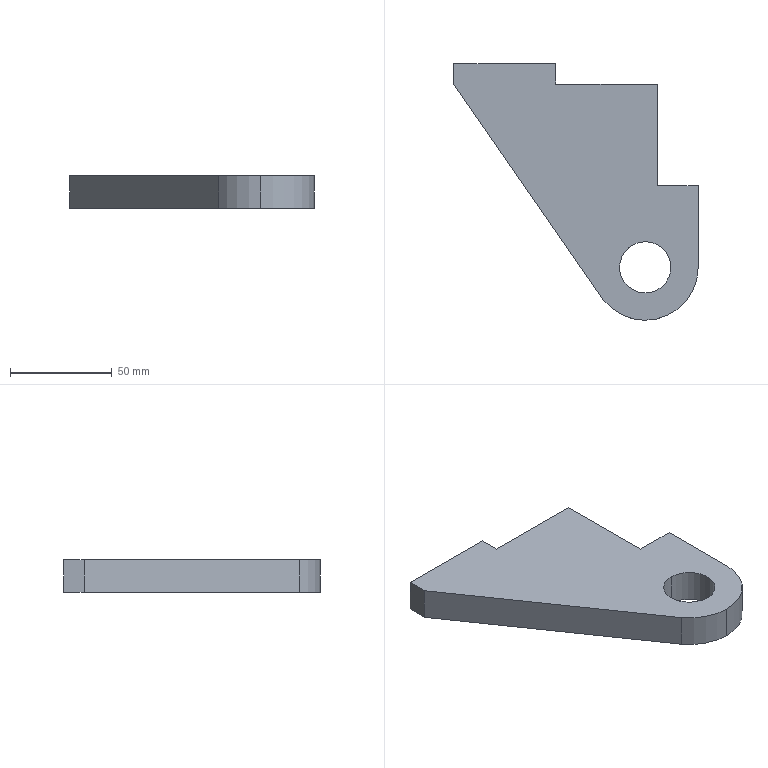Component | SolidWorks | VehicleBodyUpperLug-2 | 1 solid | 14 faces | box 120 x 126 x 16 mm | volume 129354 mm3 | plane 10 | cylinder 4 | commonest cylinder face diameters 25.2 x2 52 x2 | material Q235
build123d program:
from build123d import *

# Parameters (mm, degrees)
SKETCH1_R           = 12.6
BOSS_EXTRUDE1_DEPTH = 16


with BuildPart() as part:
    # Sketch1 → Boss-Extrude1 (new body)
    with BuildSketch(Plane.XY):
        with BuildLine():
            Line((96.756, 48.198), (133.752, 48.562))
            Line((133.752, 48.562), (133.556, 68.561))
            Line((133.556, 68.561), (183.553, 69.052))
            Line((183.553, 69.052), (183.259, 99.05))
            Line((183.259, 99.05), (183.062, 119.049))
            Line((183.062, 119.049), (193.062, 119.147))
            Line((193.062, 119.147), (192.571, 169.145))
            Line((192.571, 169.145), (182.571, 169.047))
            Line((182.571, 169.047), (77.704, 94.818))
            ThreePointArc((77.704, 94.818), (68.916, 65.708), (93.756, 48.169))
            Line((93.756, 48.169), (96.756, 48.198))
        make_face()
        with Locations((93.501, 74.168)):
            Circle(SKETCH1_R, mode=Mode.SUBTRACT)
    extrude(amount=BOSS_EXTRUDE1_DEPTH)


solid = part.part

# Placed as in the assembly
solid = solid.moved(Location((-209.351, 1092.251, 2619.537), (0, 0, 89.437)))
STEP:
#1=COLOUR_RGB('',0.7922,0.8196,0.9333);
#2=FILL_AREA_STYLE_COLOUR('',#1);
#3=FILL_AREA_STYLE('',(#2));
#4=SURFACE_STYLE_FILL_AREA(#3);
#5=SURFACE_SIDE_STYLE('',(#4));
#6=SURFACE_STYLE_USAGE(.BOTH.,#5);
#7=PRESENTATION_STYLE_ASSIGNMENT((#6));
#8=CARTESIAN_POINT('',(-11.131,46.216,103.761));
#9=VERTEX_POINT('',#8);
#10=CARTESIAN_POINT('',(-11.121,47.208,103.761));
#11=VERTEX_POINT('',#10);
#12=CARTESIAN_POINT('',(-11.126,46.712,103.761));
#13=DIRECTION('',(0.,0.,1.));
#14=DIRECTION('',(0.009819,1.,0.));
#15=AXIS2_PLACEMENT_3D('',#12,#13,#14);
#16=CIRCLE('',#15,0.4961);
#17=EDGE_CURVE('',#9,#11,#16,.T.);
#18=ORIENTED_EDGE('',*,*,#17,.T.);
#19=CARTESIAN_POINT('',(-11.121,47.208,103.131));
#20=VERTEX_POINT('',#19);
#21=CARTESIAN_POINT('',(-11.121,47.208,103.761));
#22=DIRECTION('',(-0.,-0.,-1.));
#23=VECTOR('',#22,39.37);
#24=LINE('',#21,#23);
#25=EDGE_CURVE('',#11,#20,#24,.T.);
#26=ORIENTED_EDGE('',*,*,#25,.T.);
#27=CARTESIAN_POINT('',(-11.131,46.216,103.131));
#28=VERTEX_POINT('',#27);
#29=CARTESIAN_POINT('',(-11.126,46.712,103.131));
#30=DIRECTION('',(0.,0.,1.));
#31=DIRECTION('',(0.009819,1.,0.));
#32=AXIS2_PLACEMENT_3D('',#29,#30,#31);
#33=CIRCLE('',#32,0.4961);
#34=EDGE_CURVE('',#28,#20,#33,.T.);
#35=ORIENTED_EDGE('',*,*,#34,.F.);
#36=CARTESIAN_POINT('',(-11.131,46.216,103.761));
#37=DIRECTION('',(-0.,-0.,-1.));
#38=VECTOR('',#37,39.37);
#39=LINE('',#36,#38);
#40=EDGE_CURVE('',#9,#28,#39,.T.);
#41=ORIENTED_EDGE('',*,*,#40,.F.);
#42=EDGE_LOOP('',(#18,#26,#35,#41));
#43=FACE_OUTER_BOUND('',#42,.T.);
#44=CARTESIAN_POINT('',(-11.126,46.712,103.761));
#45=DIRECTION('',(-0.,-0.,-1.));
#46=DIRECTION('',(-0.009819,-1.,0.));
#47=AXIS2_PLACEMENT_3D('',#44,#45,#46);
#48=CYLINDRICAL_SURFACE('',#47,0.4961);
#49=ADVANCED_FACE('',(#43),#48,.F.);
#50=CARTESIAN_POINT('',(-11.136,45.688,103.761));
#51=VERTEX_POINT('',#50);
#52=CARTESIAN_POINT('',(-10.102,46.712,103.761));
#53=VERTEX_POINT('',#52);
#54=CARTESIAN_POINT('',(-11.126,46.712,103.761));
#55=DIRECTION('',(0.,0.,1.));
#56=DIRECTION('',(0.009819,1.,0.));
#57=AXIS2_PLACEMENT_3D('',#54,#55,#56);
#58=CIRCLE('',#57,1.024);
#59=EDGE_CURVE('',#51,#53,#58,.T.);
#60=ORIENTED_EDGE('',*,*,#59,.F.);
#61=CARTESIAN_POINT('',(-11.136,45.688,103.131));
#62=VERTEX_POINT('',#61);
#63=CARTESIAN_POINT('',(-11.136,45.688,103.761));
#64=DIRECTION('',(-0.,-0.,-1.));
#65=VECTOR('',#64,39.37);
#66=LINE('',#63,#65);
#67=EDGE_CURVE('',#51,#62,#66,.T.);
#68=ORIENTED_EDGE('',*,*,#67,.T.);
#69=CARTESIAN_POINT('',(-10.102,46.712,103.131));
#70=VERTEX_POINT('',#69);
#71=CARTESIAN_POINT('',(-11.126,46.712,103.131));
#72=DIRECTION('',(0.,0.,1.));
#73=DIRECTION('',(0.009819,1.,0.));
#74=AXIS2_PLACEMENT_3D('',#71,#72,#73);
#75=CIRCLE('',#74,1.024);
#76=EDGE_CURVE('',#62,#70,#75,.T.);
#77=ORIENTED_EDGE('',*,*,#76,.T.);
#78=CARTESIAN_POINT('',(-10.102,46.712,103.761));
#79=DIRECTION('',(-0.,-0.,-1.));
#80=VECTOR('',#79,39.37);
#81=LINE('',#78,#80);
#82=EDGE_CURVE('',#53,#70,#81,.T.);
#83=ORIENTED_EDGE('',*,*,#82,.F.);
#84=EDGE_LOOP('',(#60,#68,#77,#83));
#85=FACE_OUTER_BOUND('',#84,.T.);
#86=CARTESIAN_POINT('',(-11.126,46.712,103.761));
#87=DIRECTION('',(-0.,-0.,-1.));
#88=DIRECTION('',(-0.009819,-1.,0.));
#89=AXIS2_PLACEMENT_3D('',#86,#87,#88);
#90=CYLINDRICAL_SURFACE('',#89,1.024);
#91=ADVANCED_FACE('',(#85),#90,.T.);
#92=CARTESIAN_POINT('',(-11.945,46.098,103.131));
#93=VERTEX_POINT('',#92);
#94=CARTESIAN_POINT('',(-14.827,50.255,103.131));
#95=VERTEX_POINT('',#94);
#96=CARTESIAN_POINT('',(-9.294,42.273,103.131));
#97=DIRECTION('',(-0.5697,0.8219,0.));
#98=VECTOR('',#97,39.37);
#99=LINE('',#96,#98);
#100=EDGE_CURVE('',#93,#95,#99,.T.);
#101=ORIENTED_EDGE('',*,*,#100,.F.);
#102=CARTESIAN_POINT('',(-11.945,46.098,103.761));
#103=VERTEX_POINT('',#102);
#104=CARTESIAN_POINT('',(-11.945,46.098,103.761));
#105=DIRECTION('',(-0.,-0.,-1.));
#106=VECTOR('',#105,39.37);
#107=LINE('',#104,#106);
#108=EDGE_CURVE('',#103,#93,#107,.T.);
#109=ORIENTED_EDGE('',*,*,#108,.F.);
#110=CARTESIAN_POINT('',(-14.827,50.255,103.761));
#111=VERTEX_POINT('',#110);
#112=CARTESIAN_POINT('',(-9.294,42.273,103.761));
#113=DIRECTION('',(-0.5697,0.8219,0.));
#114=VECTOR('',#113,39.37);
#115=LINE('',#112,#114);
#116=EDGE_CURVE('',#103,#111,#115,.T.);
#117=ORIENTED_EDGE('',*,*,#116,.T.);
#118=CARTESIAN_POINT('',(-14.827,50.255,103.761));
#119=DIRECTION('',(-0.,-0.,-1.));
#120=VECTOR('',#119,39.37);
#121=LINE('',#118,#120);
#122=EDGE_CURVE('',#111,#95,#121,.T.);
#123=ORIENTED_EDGE('',*,*,#122,.T.);
#124=EDGE_LOOP('',(#101,#109,#117,#123));
#125=FACE_OUTER_BOUND('',#124,.T.);
#126=CARTESIAN_POINT('',(-9.294,42.273,103.761));
#127=DIRECTION('',(-0.8219,-0.5697,0.));
#128=DIRECTION('',(0.5697,-0.8219,-0.));
#129=AXIS2_PLACEMENT_3D('',#126,#127,#128);
#130=PLANE('',#129);
#131=ADVANCED_FACE('',(#125),#130,.T.);
#132=ORIENTED_EDGE('',*,*,#67,.F.);
#133=CARTESIAN_POINT('',(-11.126,46.712,103.761));
#134=DIRECTION('',(0.,0.,1.));
#135=DIRECTION('',(0.009819,1.,0.));
#136=AXIS2_PLACEMENT_3D('',#133,#134,#135);
#137=CIRCLE('',#136,1.024);
#138=EDGE_CURVE('',#103,#51,#137,.T.);
#139=ORIENTED_EDGE('',*,*,#138,.F.);
#140=ORIENTED_EDGE('',*,*,#108,.T.);
#141=CARTESIAN_POINT('',(-11.126,46.712,103.131));
#142=DIRECTION('',(0.,0.,1.));
#143=DIRECTION('',(0.009819,1.,0.));
#144=AXIS2_PLACEMENT_3D('',#141,#142,#143);
#145=CIRCLE('',#144,1.024);
#146=EDGE_CURVE('',#93,#62,#145,.T.);
#147=ORIENTED_EDGE('',*,*,#146,.T.);
#148=EDGE_LOOP('',(#132,#139,#140,#147));
#149=FACE_OUTER_BOUND('',#148,.T.);
#150=CARTESIAN_POINT('',(-11.126,46.712,103.761));
#151=DIRECTION('',(-0.,-0.,-1.));
#152=DIRECTION('',(-0.009819,-1.,0.));
#153=AXIS2_PLACEMENT_3D('',#150,#151,#152);
#154=CYLINDRICAL_SURFACE('',#153,1.024);
#155=ADVANCED_FACE('',(#149),#154,.T.);
#156=CARTESIAN_POINT('',(-10.102,48.286,103.131));
#157=VERTEX_POINT('',#156);
#158=CARTESIAN_POINT('',(-10.102,43.002,103.131));
#159=DIRECTION('',(-0.,1.,-0.));
#160=VECTOR('',#159,39.37);
#161=LINE('',#158,#160);
#162=EDGE_CURVE('',#70,#157,#161,.T.);
#163=ORIENTED_EDGE('',*,*,#162,.T.);
#164=CARTESIAN_POINT('',(-10.102,48.286,103.761));
#165=VERTEX_POINT('',#164);
#166=CARTESIAN_POINT('',(-10.102,48.286,103.761));
#167=DIRECTION('',(-0.,-0.,-1.));
#168=VECTOR('',#167,39.37);
#169=LINE('',#166,#168);
#170=EDGE_CURVE('',#165,#157,#169,.T.);
#171=ORIENTED_EDGE('',*,*,#170,.F.);
#172=CARTESIAN_POINT('',(-10.102,43.002,103.761));
#173=DIRECTION('',(-0.,1.,-0.));
#174=VECTOR('',#173,39.37);
#175=LINE('',#172,#174);
#176=EDGE_CURVE('',#53,#165,#175,.T.);
#177=ORIENTED_EDGE('',*,*,#176,.F.);
#178=ORIENTED_EDGE('',*,*,#82,.T.);
#179=EDGE_LOOP('',(#163,#171,#177,#178));
#180=FACE_OUTER_BOUND('',#179,.T.);
#181=CARTESIAN_POINT('',(-10.102,43.002,103.761));
#182=DIRECTION('',(-1.,-0.,0.));
#183=DIRECTION('',(0.,-1.,0.));
#184=AXIS2_PLACEMENT_3D('',#181,#182,#183);
#185=PLANE('',#184);
#186=ADVANCED_FACE('',(#180),#185,.F.);
#187=CARTESIAN_POINT('',(-10.89,48.286,103.131));
#188=VERTEX_POINT('',#187);
#189=CARTESIAN_POINT('',(-8.242,48.286,103.131));
#190=DIRECTION('',(-1.,0.,0.));
#191=VECTOR('',#190,39.37);
#192=LINE('',#189,#191);
#193=EDGE_CURVE('',#157,#188,#192,.T.);
#194=ORIENTED_EDGE('',*,*,#193,.T.);
#195=CARTESIAN_POINT('',(-10.89,48.286,103.761));
#196=VERTEX_POINT('',#195);
#197=CARTESIAN_POINT('',(-10.89,48.286,103.761));
#198=DIRECTION('',(-0.,-0.,-1.));
#199=VECTOR('',#198,39.37);
#200=LINE('',#197,#199);
#201=EDGE_CURVE('',#196,#188,#200,.T.);
#202=ORIENTED_EDGE('',*,*,#201,.F.);
#203=CARTESIAN_POINT('',(-8.242,48.286,103.761));
#204=DIRECTION('',(-1.,0.,0.));
#205=VECTOR('',#204,39.37);
#206=LINE('',#203,#205);
#207=EDGE_CURVE('',#165,#196,#206,.T.);
#208=ORIENTED_EDGE('',*,*,#207,.F.);
#209=ORIENTED_EDGE('',*,*,#170,.T.);
#210=EDGE_LOOP('',(#194,#202,#208,#209));
#211=FACE_OUTER_BOUND('',#210,.T.);
#212=CARTESIAN_POINT('',(-8.242,48.286,103.761));
#213=DIRECTION('',(-0.,-1.,0.));
#214=DIRECTION('',(1.,-0.,-0.));
#215=AXIS2_PLACEMENT_3D('',#212,#213,#214);
#216=PLANE('',#215);
#217=ADVANCED_FACE('',(#211),#216,.F.);
#218=CARTESIAN_POINT('',(-10.89,50.255,103.131));
#219=VERTEX_POINT('',#218);
#220=CARTESIAN_POINT('',(-10.89,43.002,103.131));
#221=DIRECTION('',(0.,1.,-0.));
#222=VECTOR('',#221,39.37);
#223=LINE('',#220,#222);
#224=EDGE_CURVE('',#188,#219,#223,.T.);
#225=ORIENTED_EDGE('',*,*,#224,.T.);
#226=CARTESIAN_POINT('',(-10.89,50.255,103.761));
#227=VERTEX_POINT('',#226);
#228=CARTESIAN_POINT('',(-10.89,50.255,103.761));
#229=DIRECTION('',(-0.,-0.,-1.));
#230=VECTOR('',#229,39.37);
#231=LINE('',#228,#230);
#232=EDGE_CURVE('',#227,#219,#231,.T.);
#233=ORIENTED_EDGE('',*,*,#232,.F.);
#234=CARTESIAN_POINT('',(-10.89,43.002,103.761));
#235=DIRECTION('',(0.,1.,-0.));
#236=VECTOR('',#235,39.37);
#237=LINE('',#234,#236);
#238=EDGE_CURVE('',#196,#227,#237,.T.);
#239=ORIENTED_EDGE('',*,*,#238,.F.);
#240=ORIENTED_EDGE('',*,*,#201,.T.);
#241=EDGE_LOOP('',(#225,#233,#239,#240));
#242=FACE_OUTER_BOUND('',#241,.T.);
#243=CARTESIAN_POINT('',(-10.89,43.002,103.761));
#244=DIRECTION('',(-1.,0.,0.));
#245=DIRECTION('',(-0.,-1.,0.));
#246=AXIS2_PLACEMENT_3D('',#243,#244,#245);
#247=PLANE('',#246);
#248=ADVANCED_FACE('',(#242),#247,.F.);
#249=CARTESIAN_POINT('',(-12.858,50.255,103.131));
#250=VERTEX_POINT('',#249);
#251=CARTESIAN_POINT('',(-8.242,50.255,103.131));
#252=DIRECTION('',(1.,0.,-0.));
#253=VECTOR('',#252,39.37);
#254=LINE('',#251,#253);
#255=EDGE_CURVE('',#250,#219,#254,.T.);
#256=ORIENTED_EDGE('',*,*,#255,.F.);
#257=CARTESIAN_POINT('',(-12.858,50.255,103.761));
#258=VERTEX_POINT('',#257);
#259=CARTESIAN_POINT('',(-12.858,50.255,103.761));
#260=DIRECTION('',(-0.,-0.,-1.));
#261=VECTOR('',#260,39.37);
#262=LINE('',#259,#261);
#263=EDGE_CURVE('',#258,#250,#262,.T.);
#264=ORIENTED_EDGE('',*,*,#263,.F.);
#265=CARTESIAN_POINT('',(-8.242,50.255,103.761));
#266=DIRECTION('',(1.,0.,-0.));
#267=VECTOR('',#266,39.37);
#268=LINE('',#265,#267);
#269=EDGE_CURVE('',#258,#227,#268,.T.);
#270=ORIENTED_EDGE('',*,*,#269,.T.);
#271=ORIENTED_EDGE('',*,*,#232,.T.);
#272=EDGE_LOOP('',(#256,#264,#270,#271));
#273=FACE_OUTER_BOUND('',#272,.T.);
#274=CARTESIAN_POINT('',(-8.242,50.255,103.761));
#275=DIRECTION('',(-0.,1.,-0.));
#276=DIRECTION('',(-1.,-0.,0.));
#277=AXIS2_PLACEMENT_3D('',#274,#275,#276);
#278=PLANE('',#277);
#279=ADVANCED_FACE('',(#273),#278,.T.);
#280=CARTESIAN_POINT('',(-12.858,50.649,103.131));
#281=VERTEX_POINT('',#280);
#282=CARTESIAN_POINT('',(-12.858,43.002,103.131));
#283=DIRECTION('',(0.,1.,-0.));
#284=VECTOR('',#283,39.37);
#285=LINE('',#282,#284);
#286=EDGE_CURVE('',#250,#281,#285,.T.);
#287=ORIENTED_EDGE('',*,*,#286,.T.);
#288=CARTESIAN_POINT('',(-12.858,50.649,103.761));
#289=VERTEX_POINT('',#288);
#290=CARTESIAN_POINT('',(-12.858,50.649,103.761));
#291=DIRECTION('',(-0.,-0.,-1.));
#292=VECTOR('',#291,39.37);
#293=LINE('',#290,#292);
#294=EDGE_CURVE('',#289,#281,#293,.T.);
#295=ORIENTED_EDGE('',*,*,#294,.F.);
#296=CARTESIAN_POINT('',(-12.858,43.002,103.761));
#297=DIRECTION('',(0.,1.,-0.));
#298=VECTOR('',#297,39.37);
#299=LINE('',#296,#298);
#300=EDGE_CURVE('',#258,#289,#299,.T.);
#301=ORIENTED_EDGE('',*,*,#300,.F.);
#302=ORIENTED_EDGE('',*,*,#263,.T.);
#303=EDGE_LOOP('',(#287,#295,#301,#302));
#304=FACE_OUTER_BOUND('',#303,.T.);
#305=CARTESIAN_POINT('',(-12.858,43.002,103.761));
#306=DIRECTION('',(-1.,0.,0.));
#307=DIRECTION('',(-0.,-1.,0.));
#308=AXIS2_PLACEMENT_3D('',#305,#306,#307);
#309=PLANE('',#308);
#310=ADVANCED_FACE('',(#304),#309,.F.);
#311=CARTESIAN_POINT('',(-14.827,50.649,103.131));
#312=VERTEX_POINT('',#311);
#313=CARTESIAN_POINT('',(-8.242,50.649,103.131));
#314=DIRECTION('',(-1.,0.,0.));
#315=VECTOR('',#314,39.37);
#316=LINE('',#313,#315);
#317=EDGE_CURVE('',#281,#312,#316,.T.);
#318=ORIENTED_EDGE('',*,*,#317,.T.);
#319=CARTESIAN_POINT('',(-14.827,50.649,103.761));
#320=VERTEX_POINT('',#319);
#321=CARTESIAN_POINT('',(-14.827,50.649,103.761));
#322=DIRECTION('',(-0.,-0.,-1.));
#323=VECTOR('',#322,39.37);
#324=LINE('',#321,#323);
#325=EDGE_CURVE('',#320,#312,#324,.T.);
#326=ORIENTED_EDGE('',*,*,#325,.F.);
#327=CARTESIAN_POINT('',(-8.242,50.649,103.761));
#328=DIRECTION('',(-1.,0.,0.));
#329=VECTOR('',#328,39.37);
#330=LINE('',#327,#329);
#331=EDGE_CURVE('',#289,#320,#330,.T.);
#332=ORIENTED_EDGE('',*,*,#331,.F.);
#333=ORIENTED_EDGE('',*,*,#294,.T.);
#334=EDGE_LOOP('',(#318,#326,#332,#333));
#335=FACE_OUTER_BOUND('',#334,.T.);
#336=CARTESIAN_POINT('',(-8.242,50.649,103.761));
#337=DIRECTION('',(-0.,-1.,0.));
#338=DIRECTION('',(1.,-0.,-0.));
#339=AXIS2_PLACEMENT_3D('',#336,#337,#338);
#340=PLANE('',#339);
#341=ADVANCED_FACE('',(#335),#340,.F.);
#342=ORIENTED_EDGE('',*,*,#25,.F.);
#343=CARTESIAN_POINT('',(-11.126,46.712,103.761));
#344=DIRECTION('',(0.,0.,1.));
#345=DIRECTION('',(0.009819,1.,0.));
#346=AXIS2_PLACEMENT_3D('',#343,#344,#345);
#347=CIRCLE('',#346,0.4961);
#348=EDGE_CURVE('',#11,#9,#347,.T.);
#349=ORIENTED_EDGE('',*,*,#348,.T.);
#350=ORIENTED_EDGE('',*,*,#40,.T.);
#351=CARTESIAN_POINT('',(-11.126,46.712,103.131));
#352=DIRECTION('',(0.,0.,1.));
#353=DIRECTION('',(0.009819,1.,0.));
#354=AXIS2_PLACEMENT_3D('',#351,#352,#353);
#355=CIRCLE('',#354,0.4961);
#356=EDGE_CURVE('',#20,#28,#355,.T.);
#357=ORIENTED_EDGE('',*,*,#356,.F.);
#358=EDGE_LOOP('',(#342,#349,#350,#357));
#359=FACE_OUTER_BOUND('',#358,.T.);
#360=CARTESIAN_POINT('',(-11.126,46.712,103.761));
#361=DIRECTION('',(-0.,-0.,-1.));
#362=DIRECTION('',(-0.009819,-1.,0.));
#363=AXIS2_PLACEMENT_3D('',#360,#361,#362);
#364=CYLINDRICAL_SURFACE('',#363,0.4961);
#365=ADVANCED_FACE('',(#359),#364,.F.);
#366=CARTESIAN_POINT('',(-14.827,43.002,103.131));
#367=DIRECTION('',(-0.,-1.,0.));
#368=VECTOR('',#367,39.37);
#369=LINE('',#366,#368);
#370=EDGE_CURVE('',#312,#95,#369,.T.);
#371=ORIENTED_EDGE('',*,*,#370,.T.);
#372=ORIENTED_EDGE('',*,*,#122,.F.);
#373=CARTESIAN_POINT('',(-14.827,43.002,103.761));
#374=DIRECTION('',(-0.,-1.,0.));
#375=VECTOR('',#374,39.37);
#376=LINE('',#373,#375);
#377=EDGE_CURVE('',#320,#111,#376,.T.);
#378=ORIENTED_EDGE('',*,*,#377,.F.);
#379=ORIENTED_EDGE('',*,*,#325,.T.);
#380=EDGE_LOOP('',(#371,#372,#378,#379));
#381=FACE_OUTER_BOUND('',#380,.T.);
#382=CARTESIAN_POINT('',(-14.827,43.002,103.761));
#383=DIRECTION('',(1.,-0.,-0.));
#384=DIRECTION('',(0.,1.,-0.));
#385=AXIS2_PLACEMENT_3D('',#382,#383,#384);
#386=PLANE('',#385);
#387=ADVANCED_FACE('',(#381),#386,.F.);
#388=ORIENTED_EDGE('',*,*,#17,.F.);
#389=ORIENTED_EDGE('',*,*,#348,.F.);
#390=EDGE_LOOP('',(#388,#389));
#391=FACE_BOUND('',#390,.T.);
#392=ORIENTED_EDGE('',*,*,#116,.F.);
#393=ORIENTED_EDGE('',*,*,#138,.T.);
#394=ORIENTED_EDGE('',*,*,#59,.T.);
#395=ORIENTED_EDGE('',*,*,#176,.T.);
#396=ORIENTED_EDGE('',*,*,#207,.T.);
#397=ORIENTED_EDGE('',*,*,#238,.T.);
#398=ORIENTED_EDGE('',*,*,#269,.F.);
#399=ORIENTED_EDGE('',*,*,#300,.T.);
#400=ORIENTED_EDGE('',*,*,#331,.T.);
#401=ORIENTED_EDGE('',*,*,#377,.T.);
#402=EDGE_LOOP('',(#392,#393,#394,#395,#396,#397,#398,#399,#400,#401));
#403=FACE_OUTER_BOUND('',#402,.T.);
#404=CARTESIAN_POINT('',(-8.242,43.002,103.761));
#405=DIRECTION('',(0.,0.,1.));
#406=DIRECTION('',(0.009819,1.,-0.));
#407=AXIS2_PLACEMENT_3D('',#404,#405,#406);
#408=PLANE('',#407);
#409=ADVANCED_FACE('',(#391,#403),#408,.T.);
#410=ORIENTED_EDGE('',*,*,#34,.T.);
#411=ORIENTED_EDGE('',*,*,#356,.T.);
#412=EDGE_LOOP('',(#410,#411));
#413=FACE_BOUND('',#412,.T.);
#414=ORIENTED_EDGE('',*,*,#100,.T.);
#415=ORIENTED_EDGE('',*,*,#370,.F.);
#416=ORIENTED_EDGE('',*,*,#317,.F.);
#417=ORIENTED_EDGE('',*,*,#286,.F.);
#418=ORIENTED_EDGE('',*,*,#255,.T.);
#419=ORIENTED_EDGE('',*,*,#224,.F.);
#420=ORIENTED_EDGE('',*,*,#193,.F.);
#421=ORIENTED_EDGE('',*,*,#162,.F.);
#422=ORIENTED_EDGE('',*,*,#76,.F.);
#423=ORIENTED_EDGE('',*,*,#146,.F.);
#424=EDGE_LOOP('',(#414,#415,#416,#417,#418,#419,#420,#421,#422,#423));
#425=FACE_OUTER_BOUND('',#424,.T.);
#426=CARTESIAN_POINT('',(-8.242,43.002,103.131));
#427=DIRECTION('',(0.,0.,1.));
#428=DIRECTION('',(0.009819,1.,-0.));
#429=AXIS2_PLACEMENT_3D('',#426,#427,#428);
#430=PLANE('',#429);
#431=ADVANCED_FACE('',(#413,#425),#430,.F.);
#432=CLOSED_SHELL('',(#49,#91,#131,#155,#186,#217,#248,#279,#310,#341,#365,#387,#409,#431));
#433=MANIFOLD_SOLID_BREP('',#432);
#434=STYLED_ITEM('',(#7),#433);
#435=(LENGTH_UNIT()NAMED_UNIT(*)SI_UNIT($,.METRE.));
#436=LENGTH_MEASURE_WITH_UNIT(LENGTH_MEASURE(0.0254),#435);
#437=DIMENSIONAL_EXPONENTS(1.,0.,0.,0.,0.,0.,0.);
#438=(CONVERSION_BASED_UNIT('',#436)LENGTH_UNIT()NAMED_UNIT(#437));
#439=UNCERTAINTY_MEASURE_WITH_UNIT(LENGTH_MEASURE(0.00001),#438,'','');
#440=(NAMED_UNIT(*)PLANE_ANGLE_UNIT()SI_UNIT($,.RADIAN.));
#441=(NAMED_UNIT(*)SI_UNIT($,.STERADIAN.)SOLID_ANGLE_UNIT());
#442=(GEOMETRIC_REPRESENTATION_CONTEXT(3)GLOBAL_UNCERTAINTY_ASSIGNED_CONTEXT((#439))GLOBAL_UNIT_ASSIGNED_CONTEXT((#438,#440,#441))REPRESENTATION_CONTEXT('',''));
#443=MECHANICAL_DESIGN_GEOMETRIC_PRESENTATION_REPRESENTATION('',(#434),#442);
#444=PRESENTATION_LAYER_ASSIGNMENT('','',(#434));
#445=CARTESIAN_POINT('',(0.,0.,0.));
#446=DIRECTION('',(0.,0.,1.));
#447=DIRECTION('',(1.,0.,0.));
#448=AXIS2_PLACEMENT_3D('',#445,#446,#447);
#449=(LENGTH_UNIT()NAMED_UNIT(*)SI_UNIT($,.METRE.));
#450=LENGTH_MEASURE_WITH_UNIT(LENGTH_MEASURE(0.0254),#449);
#451=DIMENSIONAL_EXPONENTS(1.,0.,0.,0.,0.,0.,0.);
#452=(CONVERSION_BASED_UNIT('',#450)LENGTH_UNIT()NAMED_UNIT(#451));
#453=UNCERTAINTY_MEASURE_WITH_UNIT(LENGTH_MEASURE(0.00001),#452,'','');
#454=(NAMED_UNIT(*)PLANE_ANGLE_UNIT()SI_UNIT($,.RADIAN.));
#455=(NAMED_UNIT(*)SI_UNIT($,.STERADIAN.)SOLID_ANGLE_UNIT());
#456=(GEOMETRIC_REPRESENTATION_CONTEXT(3)GLOBAL_UNCERTAINTY_ASSIGNED_CONTEXT((#453))GLOBAL_UNIT_ASSIGNED_CONTEXT((#452,#454,#455))REPRESENTATION_CONTEXT('',''));
#457=ADVANCED_BREP_SHAPE_REPRESENTATION('',(#433,#448),#456);